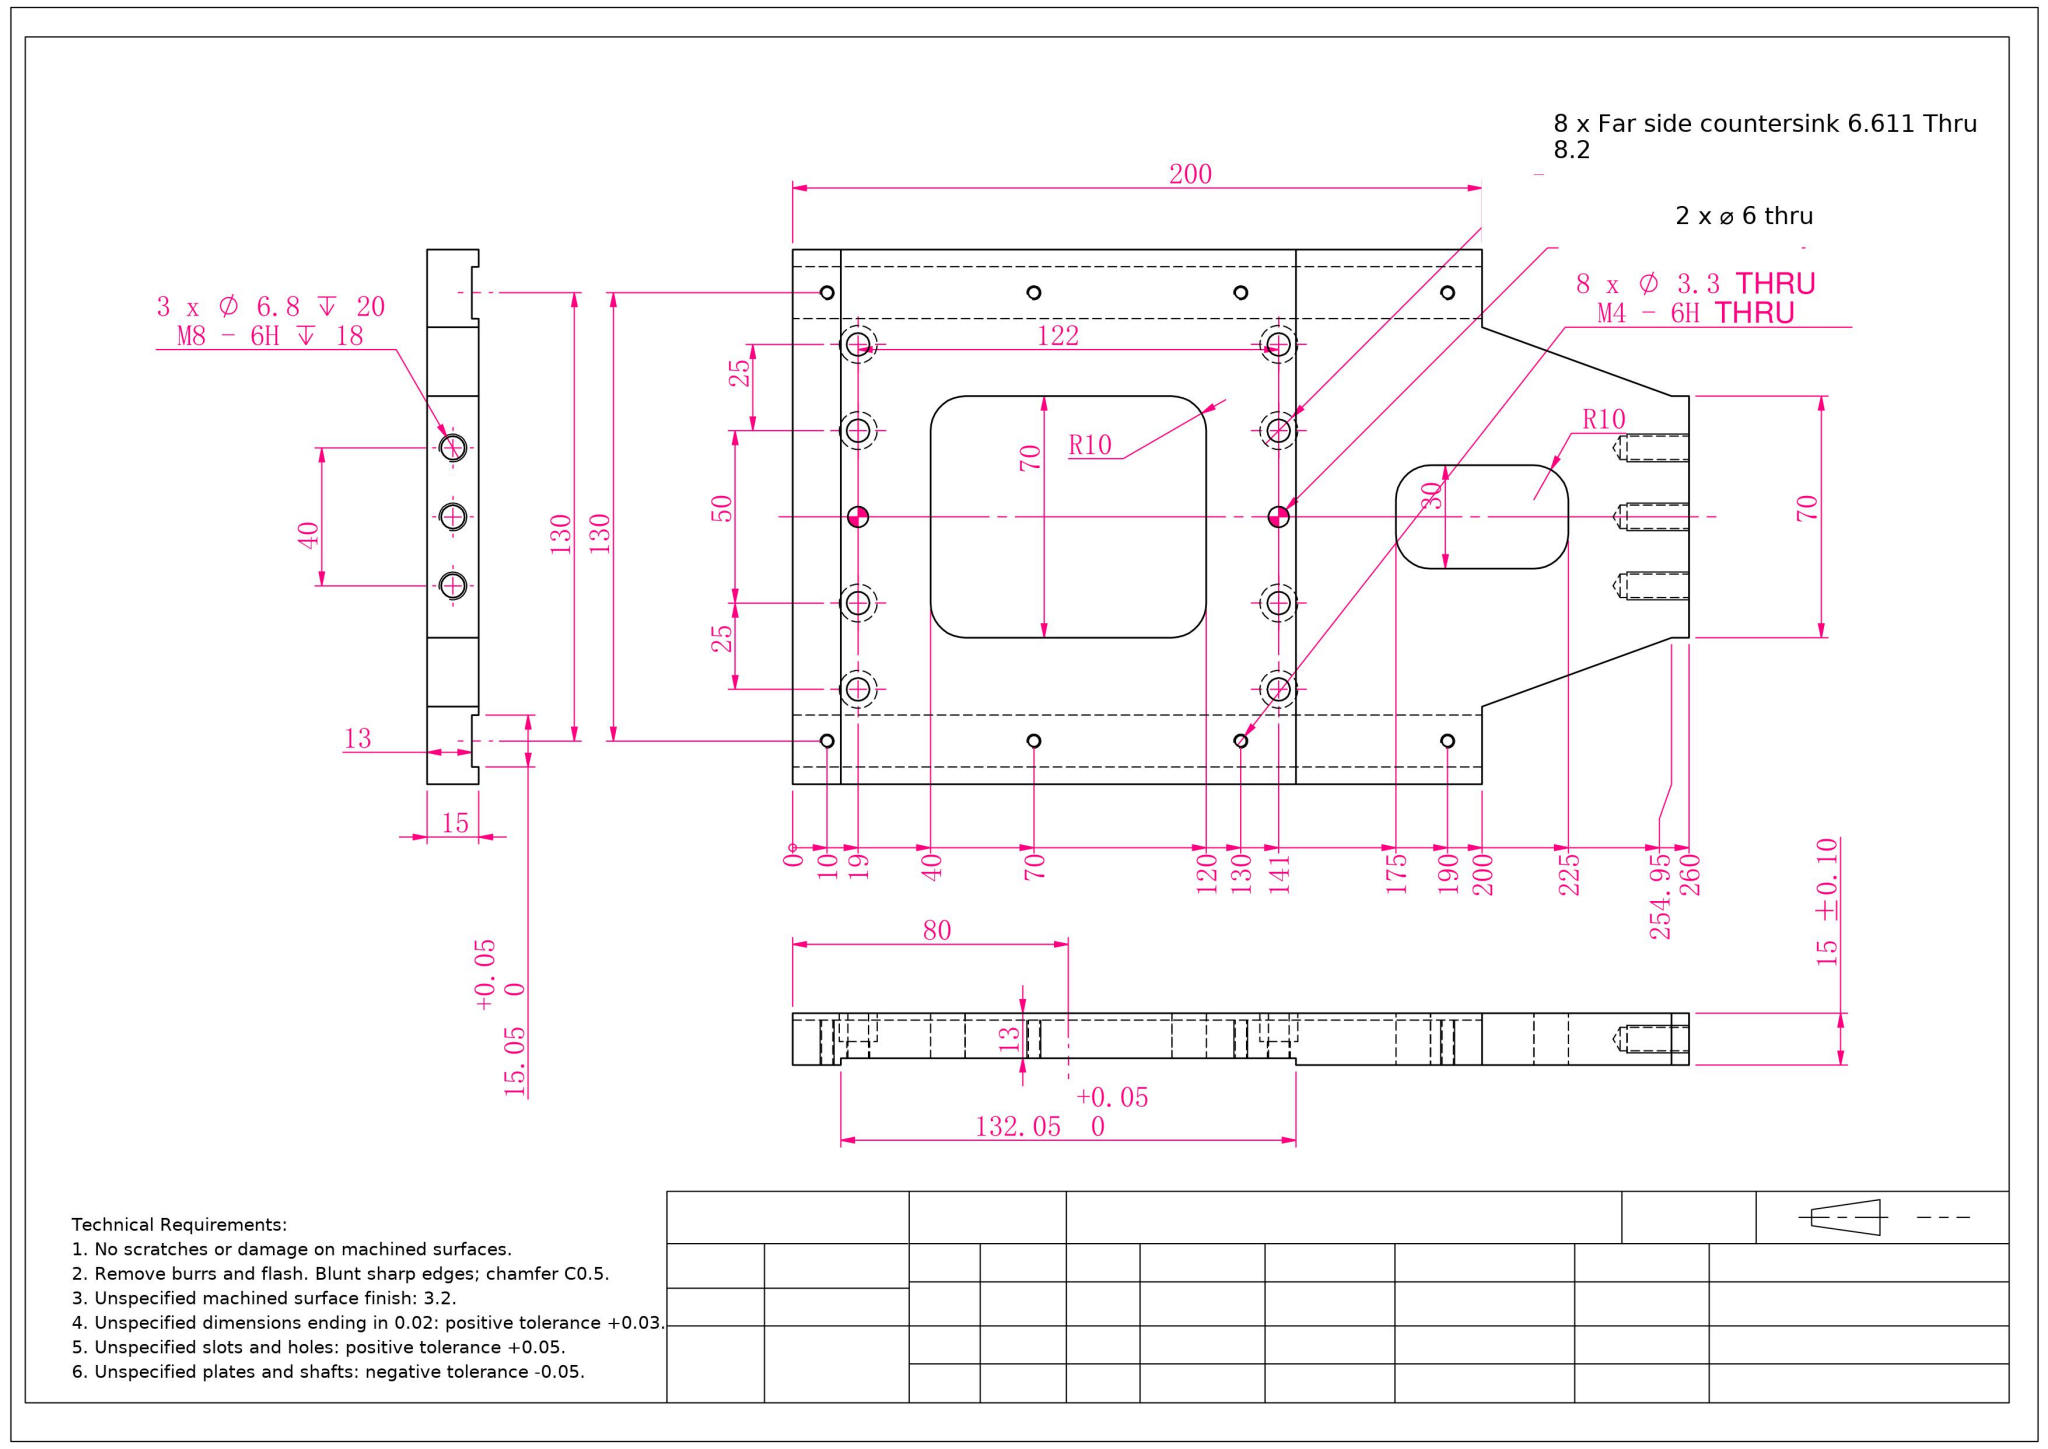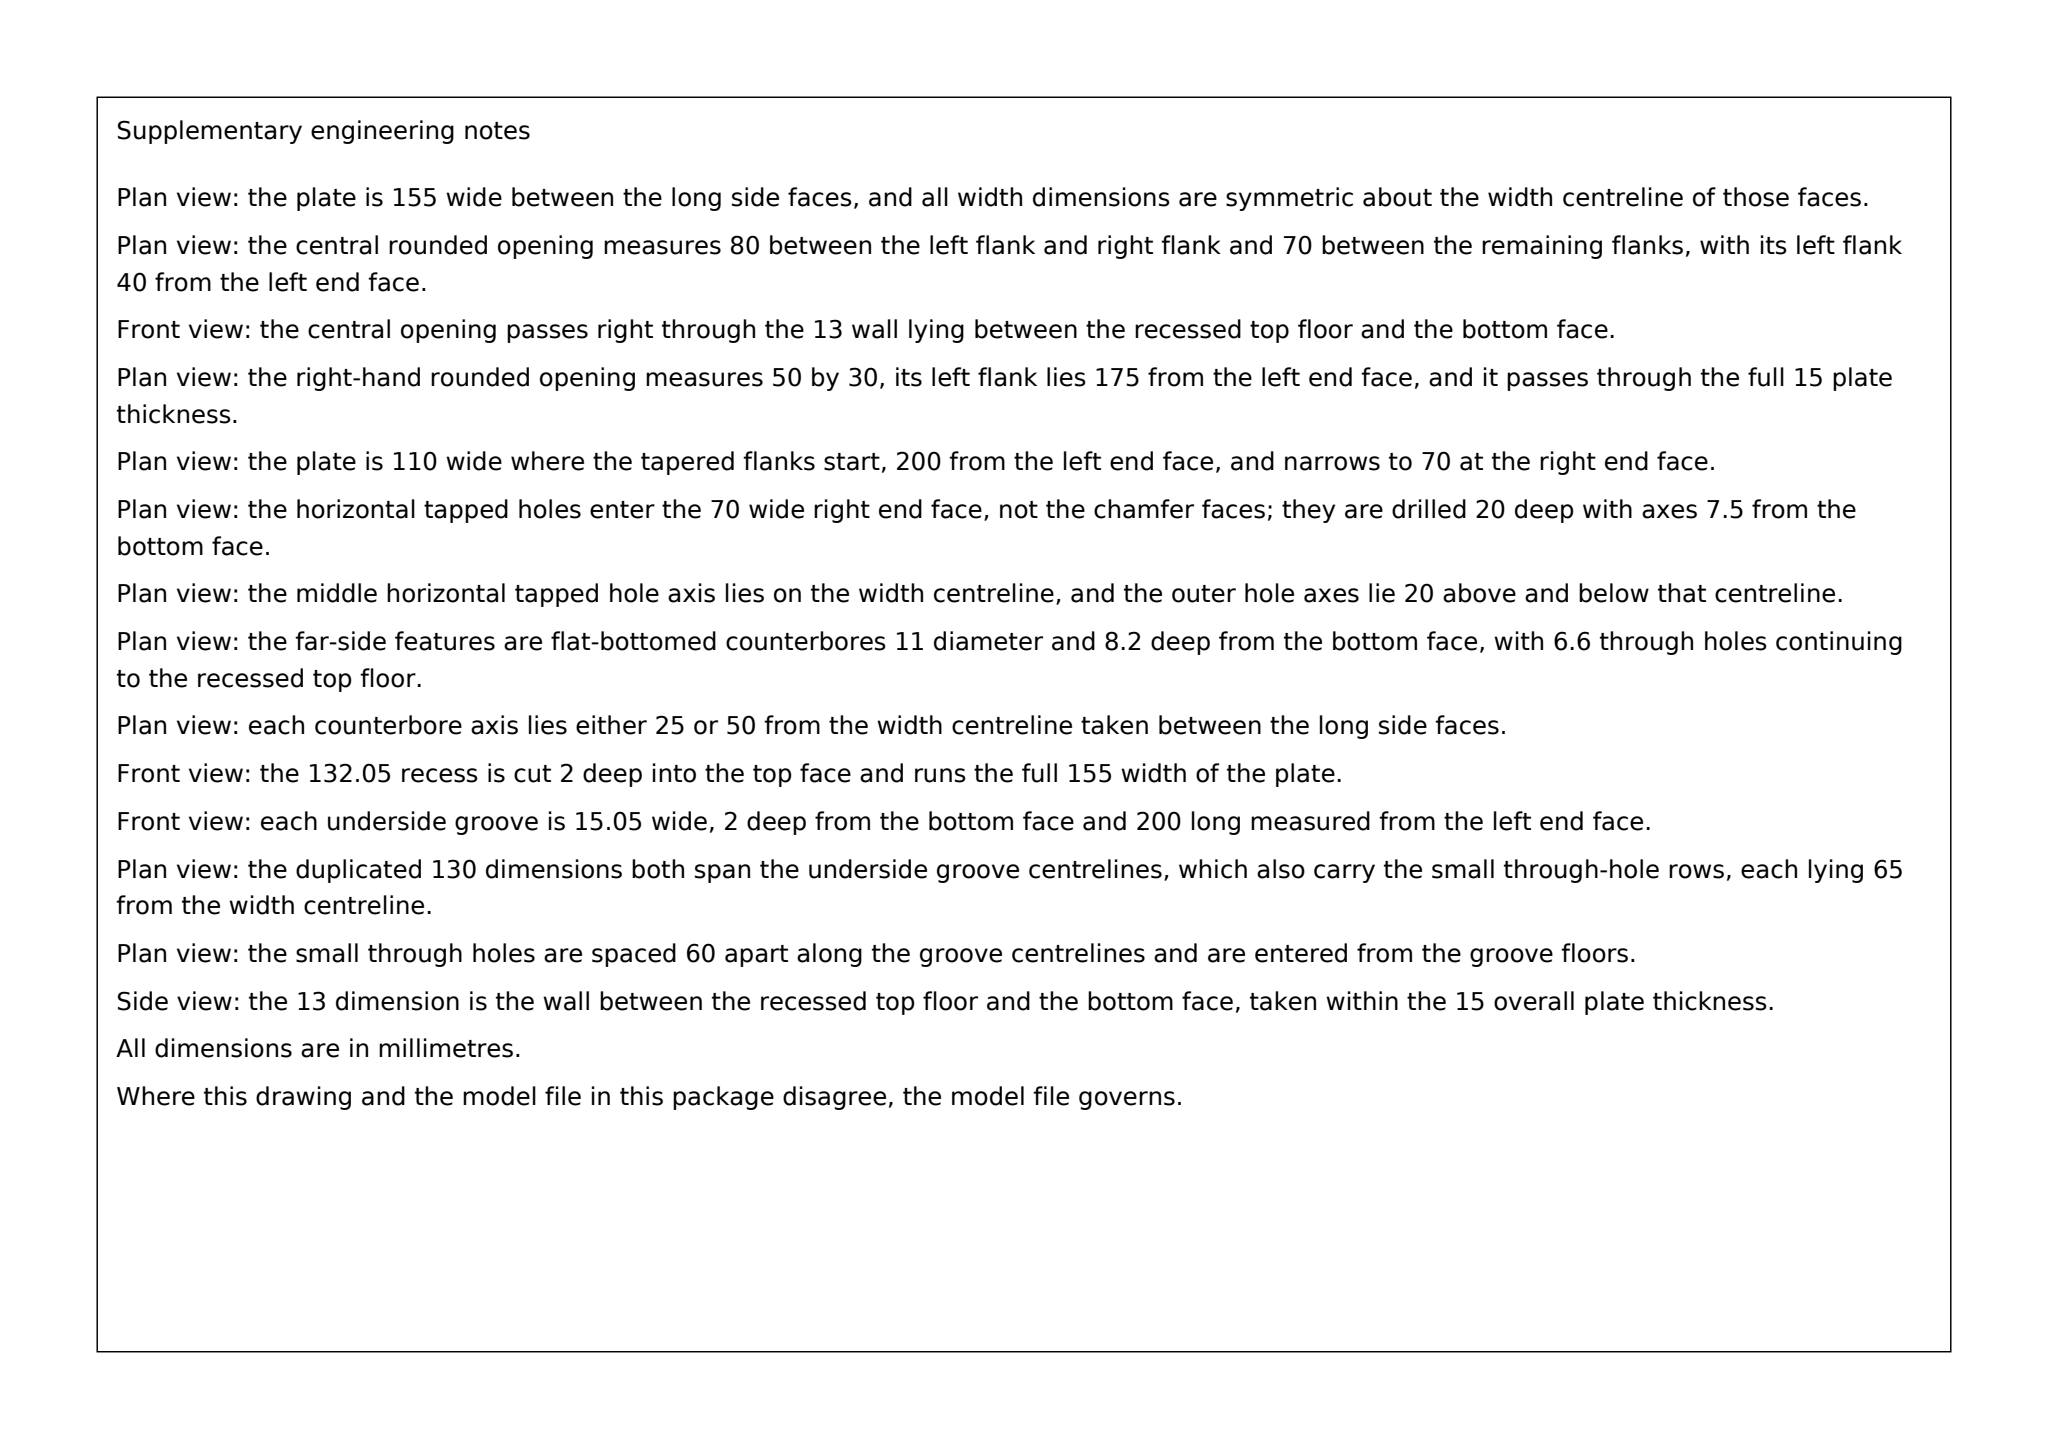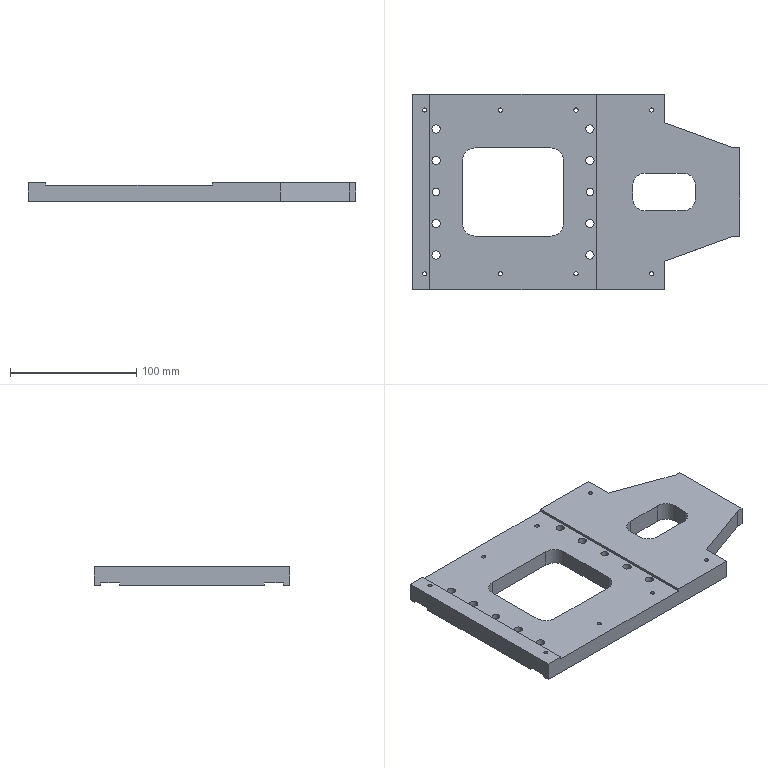Part | SolidWorks | mm | 1 solid | 112 faces | box 260 x 155 x 15 mm | volume 387256 mm3 | cylinder 66 | plane 40 | cone 6 | commonest cylinder face diameters 3.3 x16 11 x16 6.6 x16 20 x8 6.8 x6 6 x4
Drawing notes:
OVERALL 260 X 155 X 15 THK | from the solid: bbox_xyz 260 x 155 x 15
CTR POCKET 80 X 70, R10, DP 13, FLOOR Z2; X40-X120, CTR Y CL | from the solid: dia 20 (R10) z-cyls at (50,52.5)(50,102.5)(110,52.5)(110,102.5) len 13; x planes 40,120; y planes 42.5,112.5; floor z=2
RT SLOT 50 LG X 30 WD, R10, THRU; X175-X225, CTR Y CL (Y77.5) | from the solid: dia 20 z-cyls at (185,72.5)(185,82.5)(215,72.5)(215,82.5) len 15 = full thk; x planes 175,225; y planes 62.5,92.5
2X Ø6 THRU AT X19 & X141, ON Y CL (Y77.5) | from the solid: cylinders dia 6 axis z at (19,77.5) and (141,77.5), length 13 = plate thk
8X Ø6.6 THRU, Ø11 CBORE DP 8.2 FAR SIDE; X19 & X141, Y27.5/52.5/102.5/127.5 | from the solid: dia 6.6 z-cyls len 4.8 + dia 11 z-cyls len 8.2 at x=19 & 141, y=27.5/52.5/102.5/127.5; z plane 8.2
8X Ø3.3 THRU, M4-6H THRU; X10/70/130/190, Y12.5 & Y142.5 | from the solid: dia 3.3 z-cyls at x=10,70,130,190 with y=12.5 and 142.5, len 11-13 thru
3X Ø6.8 DP 20, M8-6H DP 18 IN END FACE X260; Y57.5/77.5/97.5, Z7.5 | from the solid: dia 6.8 x-axis cyls at y=57.5/77.5/97.5, z=7.5, len 20; cone 118° ref 6.8; x plane 260; thk 15
UNDERSIDE RECESS 132.05 x 15.05: STARTS 13.98 FROM LH EDGE (X0) | from the solid: x-planes 13.98 and 146.03 (146.03-13.98=132.05); y-planes 4.98/20.03 and 134.98/150.03 give 15.05 wide bands; bbox X0 = LH edge
TOP FACE EDGE RECESSES 15.05 W: RUN X0 TO X200 FROM LH EDGE | from the solid: z15 top face with z13 recess floor; x-plane 200 (2 off) terminates recesses; bbox X0 start
ALL 15.05 W EDGE RECESSES TOP & BTM FACES: 2 DP, 11 WEB | from the solid: z-planes 0/2 (btm recess) and 13/15 (top recess) = 2 deep each; 15-2-2 = 11 web, matches 11.0 long Ø3.3 holes at X70/X130
build123d program:
from build123d import *
from OCP.BRepFilletAPI import BRepFilletAPI_MakeChamfer

# Parameters (mm, degrees)
SKETCH1_W                                       = 160
SKETCH1_H                                       = 155
BOSS_EXTRUDE1_DEPTH                             = 7.5
SKETCH2_W                                       = 132.05
SKETCH2_H                                       = 155
CUT_EXTRUDE1_DEPTH                              = 2
M6_HEX_SOCKET_HEAD_CAP_SCREW_CBORE1_D           = 6.6
M6_HEX_SOCKET_HEAD_CAP_SCREW_CBORE1_CBORE_D     = 11
M6_HEX_SOCKET_HEAD_CAP_SCREW_CBORE1_CBORE_DEPTH = 8.2
SIZE_MM_DOWEL_HOLE_1_D                          = 6
BOSS_EXTRUDE2_DEPTH                             = 15
SKETCH10_W                                      = 260
SKETCH10_H                                      = 15.05
CUT_EXTRUDE2_DEPTH                              = 2
M8_TAPPED_HOLE1_D                               = 6.8
M8_TAPPED_HOLE1_DEPTH                           = 20
M8_TAPPED_HOLE1_TIP                             = 2.043
CHAMFER1_SIZE                                   = 20
CHAMFER1_SIZE2                                  = 54.95
SKETCH13_W                                      = 80
SKETCH13_H                                      = 70
SKETCH13_W_2                                    = 50
SKETCH13_H_2                                    = 30
CUT_EXTRUDE3_DEPTH                              = 197.548
FILLET1_R                                       = 10
M4_TAPPED_HOLE1_D                               = 3.3


with BuildPart() as part:
    # Sketch1 → Boss-Extrude1 (new, symmetric)
    with BuildSketch(Plane.XY):
        Rectangle(SKETCH1_W, SKETCH1_H)
    extrude(amount=BOSS_EXTRUDE1_DEPTH, both=True)

    # Sketch2 → Cut-Extrude1 (cut)
    with BuildSketch(Plane.XY.offset(7.5)):
        Rectangle(SKETCH2_W, SKETCH2_H)
    extrude(amount=-CUT_EXTRUDE1_DEPTH, mode=Mode.SUBTRACT)

    # M6 Hex Socket Head Cap Screw CBORE1 (through all)
    with Locations(Plane(origin=(0, 0, -7.5), x_dir=(-1, 0, 0), z_dir=(0, 0, -1))):
        with Locations((61, 50), (61, 25), (61, -25), (61, -50), (-61, -50), (-61, -25), (-61, 25), (-61, 50)):
            CounterBoreHole(M6_HEX_SOCKET_HEAD_CAP_SCREW_CBORE1_D / 2, M6_HEX_SOCKET_HEAD_CAP_SCREW_CBORE1_CBORE_D / 2, M6_HEX_SOCKET_HEAD_CAP_SCREW_CBORE1_CBORE_DEPTH)

    # Size mm Dowel Hole 1 (through all)
    with Locations(Plane(origin=(0, 0, -7.5), x_dir=(-1, 0, 0), z_dir=(0, 0, -1))):
        with Locations((61, 0), (-61, 0)):
            Hole(SIZE_MM_DOWEL_HOLE_1_D / 2)

    # Sketch9 → Boss-Extrude2 (add)
    with BuildSketch(Plane(origin=(0, 0, -7.5), x_dir=(-1, 0, 0), z_dir=(0, 0, -1))):
        Polygon((-180, 35), (-120, 35), (-120, 77.5), (-80, 77.5), (-80, -77.5), (-120, -77.5), (-120, -35), (-180, -35), align=None)
    extrude(amount=-BOSS_EXTRUDE2_DEPTH)

    # Sketch10 → Cut-Extrude2 (cut)
    with BuildSketch(Plane(origin=(0, 0, -7.5), x_dir=(-1, 0, 0), z_dir=(0, 0, -1))):
        with Locations((-50, 65)):
            Rectangle(SKETCH10_W, SKETCH10_H)
        with Locations((-50, -65)):
            Rectangle(SKETCH10_W, SKETCH10_H)
    extrude(amount=-CUT_EXTRUDE2_DEPTH, mode=Mode.SUBTRACT)

    # M8 Tapped Hole1
    with Locations(Plane(origin=(180, 0, 0), x_dir=(0, 0, -1), z_dir=(1, 0, 0))):
        with Locations((0, 20), (0, 0), (0, -20)):
            Hole(M8_TAPPED_HOLE1_D / 2, depth=M8_TAPPED_HOLE1_DEPTH)
            with Locations((0, 0, -(M8_TAPPED_HOLE1_DEPTH + M8_TAPPED_HOLE1_TIP / 2))):  # 118° drill point
                Cone(0, M8_TAPPED_HOLE1_D / 2, M8_TAPPED_HOLE1_TIP, mode=Mode.SUBTRACT)

    # Chamfer1: one chamfer whose edges measure the first distance from different faces: ONE call of the kernel's chamfer builder (chamfer() names one face for all edges)
    chamfer1_edges_1 = [part.edges().sort_by_distance(p)[0] for p in [
        (120, 35, 0),
    ]]
    chamfer1_side_1 = [part.faces().sort_by_distance(p)[0] for p in [
        (120, 55.816, 0.3221),
    ]]
    chamfer1_edges_2 = [part.edges().sort_by_distance(p)[0] for p in [
        (120, -35, 0),
    ]]
    chamfer1_side_2 = [part.faces().sort_by_distance(p)[0] for p in [
        (120, -55.816, 0.3221),
    ]]
    chamfer1 = BRepFilletAPI_MakeChamfer(part.part.solid().wrapped)
    for e in chamfer1_edges_1:
        chamfer1.Add(CHAMFER1_SIZE, CHAMFER1_SIZE2, e.wrapped, chamfer1_side_1[0].wrapped)  # the first distance lies on this face
    for e in chamfer1_edges_2:
        chamfer1.Add(CHAMFER1_SIZE, CHAMFER1_SIZE2, e.wrapped, chamfer1_side_2[0].wrapped)  # the first distance lies on this face
    add(Compound.cast(chamfer1.Shape()), mode=Mode.REPLACE)

    # Sketch13 → Cut-Extrude3 (cut, through all)
    with BuildSketch(Plane(origin=(0, 0, -7.5), x_dir=(-1, 0, 0), z_dir=(0, 0, -1))):
        Rectangle(SKETCH13_W, SKETCH13_H)
        with Locations((-120, 0)):
            Rectangle(SKETCH13_W_2, SKETCH13_H_2)
    extrude(amount=-CUT_EXTRUDE3_DEPTH, mode=Mode.SUBTRACT)

    # Fillet1
    fillet1_edges = [part.edges().sort_by_distance(p)[0] for p in [
        (-40, 35, -1),
        (-40, -35, -1),
        (40, -35, -1),
        (40, 35, -1),
        (145, -15, 0),
        (145, 15, 0),
        (95, 15, 0),
        (95, -15, 0),
    ]]
    fillet(fillet1_edges, radius=FILLET1_R)

    # M4 Tapped Hole1 (through all)
    with Locations(Plane(origin=(0, 0, -7.5), x_dir=(-1, 0, 0), z_dir=(0, 0, -1))):
        with Locations((70, -65), (10, -65), (-50, -65), (-110, -65), (-110, 65), (-50, 65), (10, 65), (70, 65)):
            Hole(M4_TAPPED_HOLE1_D / 2)


solid = part.part